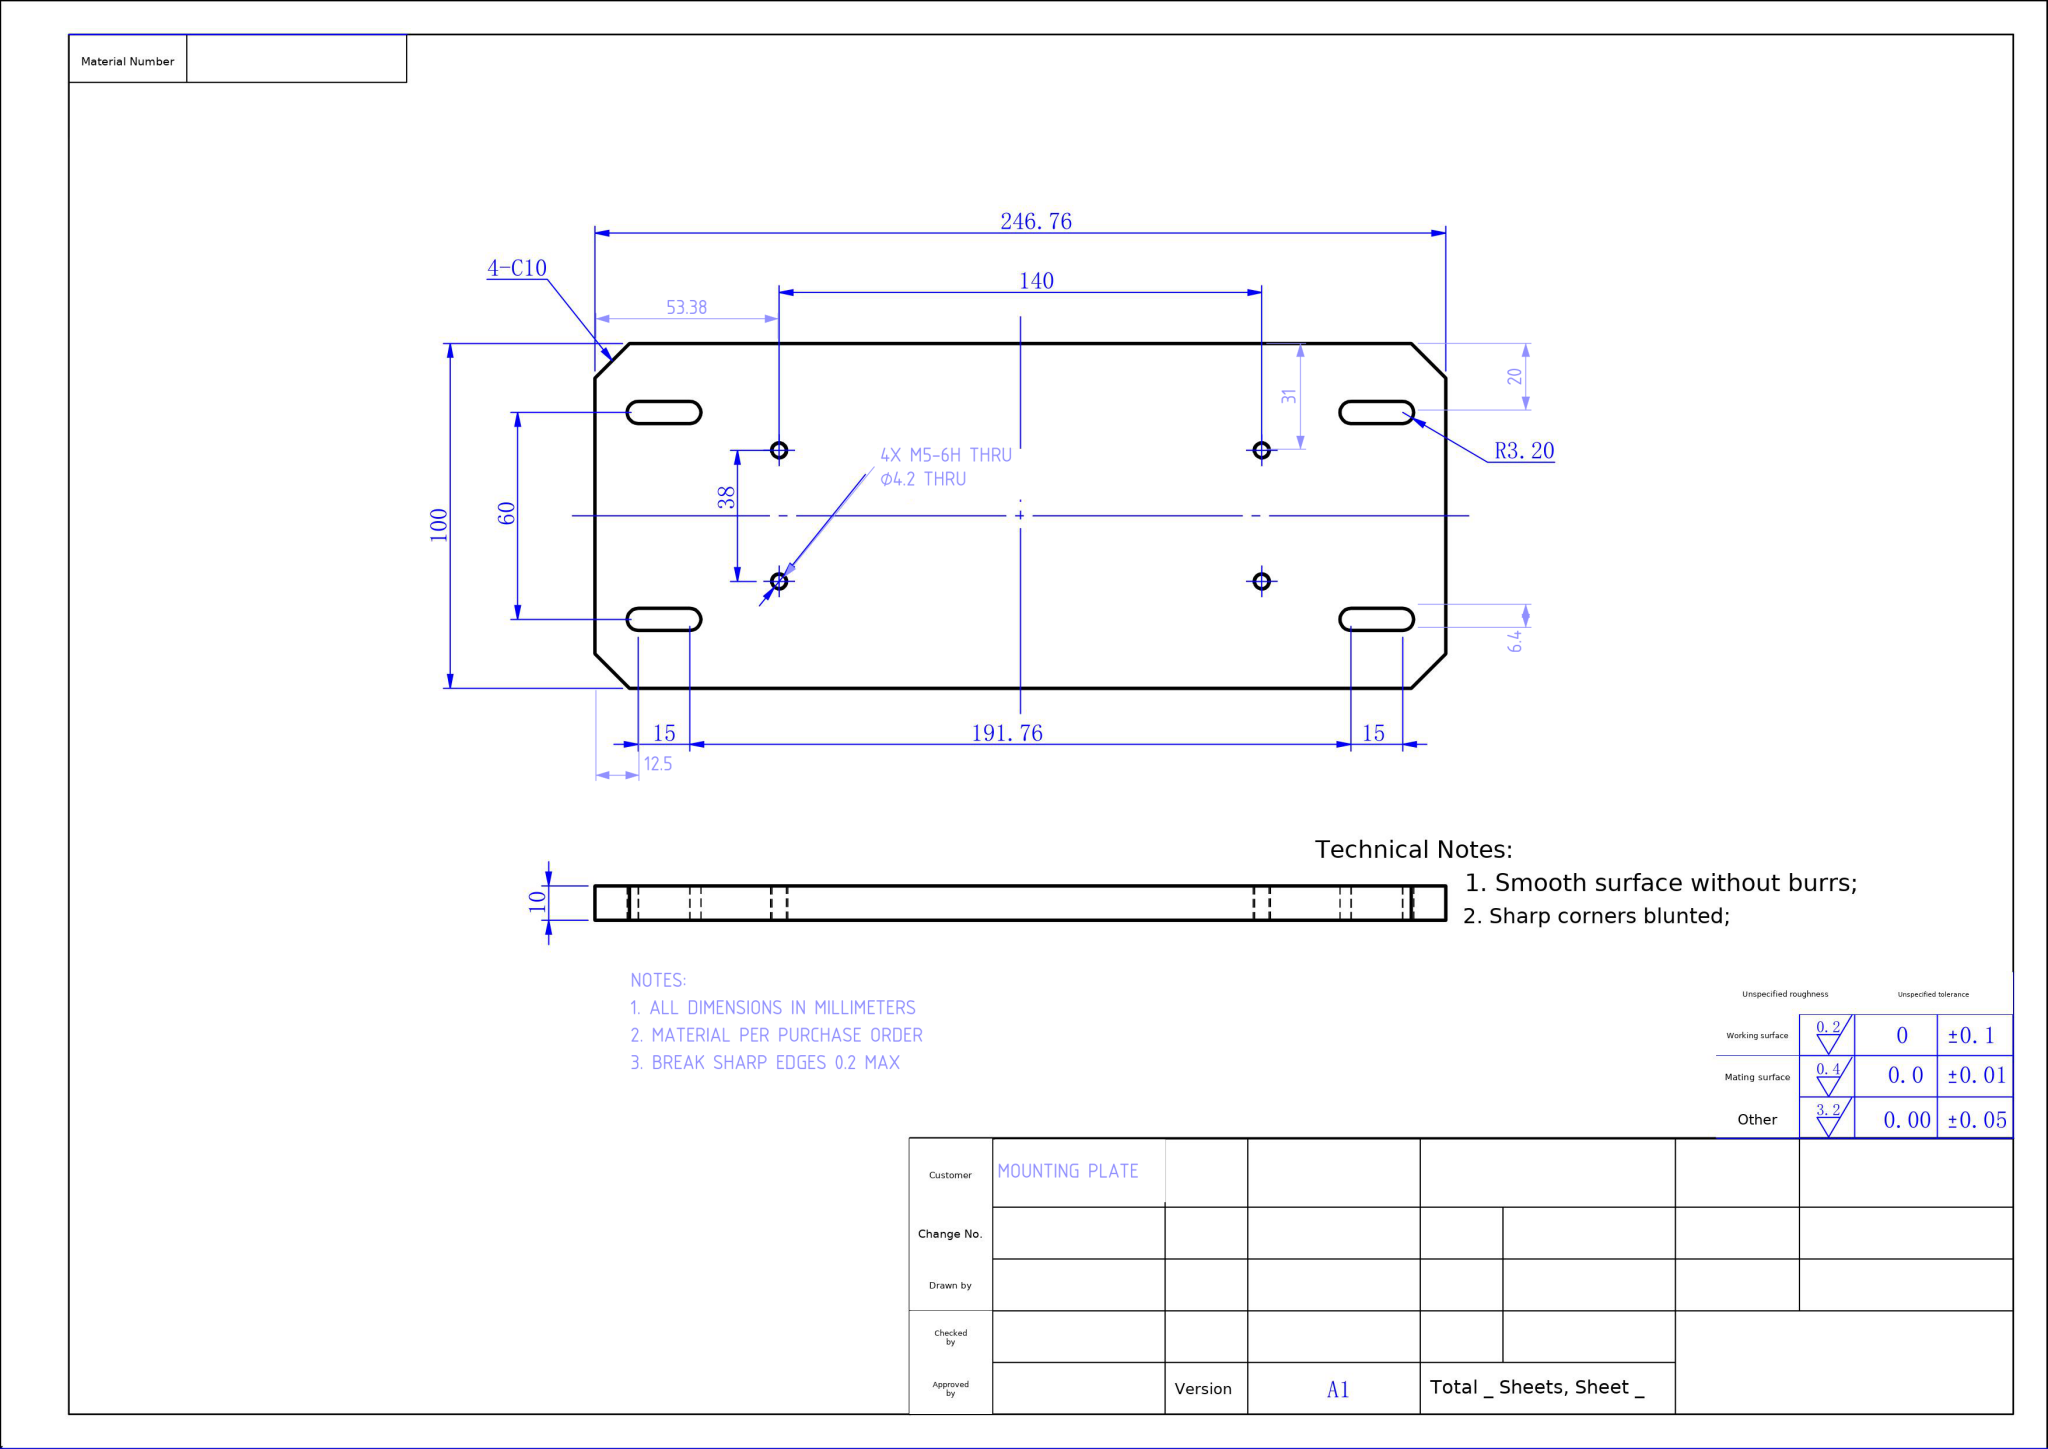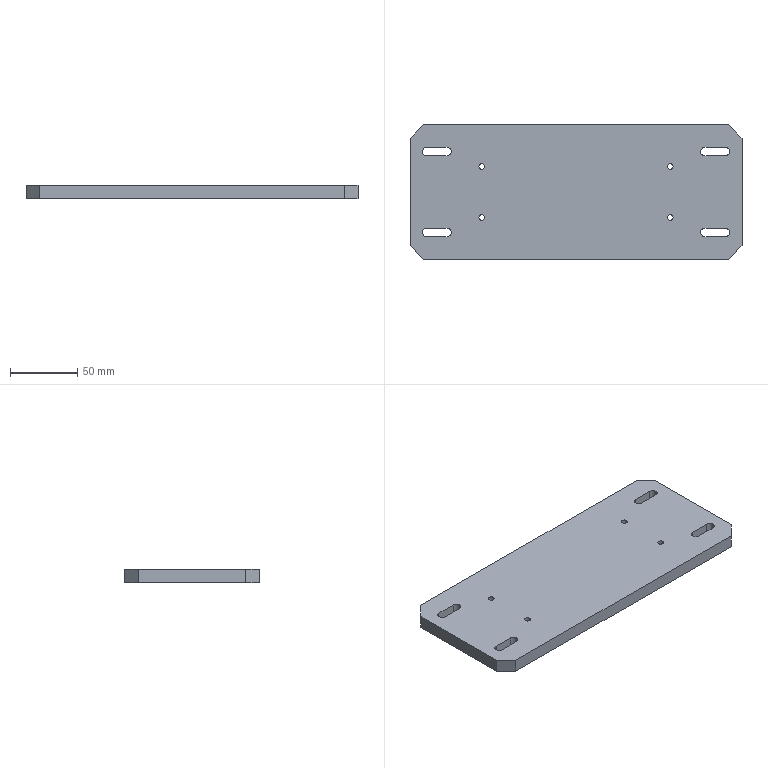Part | NX | mm | Rounded Corner Four-Slot Mounting Plate | 1 solid | 38 faces | box 246.76 x 100 x 10 mm | volume 239075 mm3 | cylinder 20 | plane 18 | commonest cylinder face diameters 6.4 x12 4.2 x8